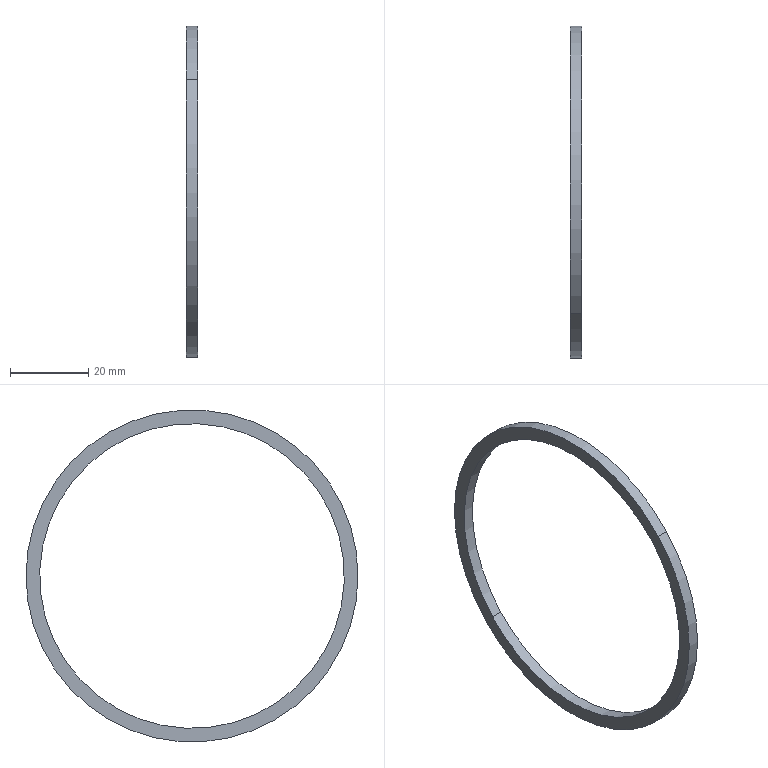Component | SolidWorks | 10BearingLockPlate-1 | 1 solid | 6 faces | box 3 x 85 x 85 mm | volume 2688 mm3 | cylinder 4 | plane 2 | commonest cylinder face diameters 78 x2 85 x2
build123d program:
from build123d import *

# Parameters (mm, degrees)
SKETCH26_R          = 42.5
SKETCH26_R_2        = 39
BOSS_EXTRUDE1_DEPTH = 3


with BuildPart() as part:
    # Sketch26 → Boss-Extrude1 (new body)
    with BuildSketch(Plane.XY):
        Circle(SKETCH26_R)
        Circle(SKETCH26_R_2, mode=Mode.SUBTRACT)
    extrude(amount=BOSS_EXTRUDE1_DEPTH)


solid = part.part

# Placed as in the assembly
solid = solid.moved(Location((210.085, -90.191, 512), (0, 90, 0)))
STEP:
#1=COLOUR_RGB('',0.7922,0.8196,0.9333);
#2=FILL_AREA_STYLE_COLOUR('',#1);
#3=FILL_AREA_STYLE('',(#2));
#4=SURFACE_STYLE_FILL_AREA(#3);
#5=SURFACE_SIDE_STYLE('',(#4));
#6=SURFACE_STYLE_USAGE(.BOTH.,#5);
#7=PRESENTATION_STYLE_ASSIGNMENT((#6));
#8=CARTESIAN_POINT('',(8.271,-2.422,19.117));
#9=VERTEX_POINT('',#8);
#10=CARTESIAN_POINT('',(8.271,-4.68,21.198));
#11=VERTEX_POINT('',#10);
#12=CARTESIAN_POINT('',(8.271,-3.551,20.157));
#13=DIRECTION('',(-1.,0.,0.));
#14=DIRECTION('',(0.,-0.7354,0.6777));
#15=AXIS2_PLACEMENT_3D('',#12,#13,#14);
#16=CIRCLE('',#15,1.535);
#17=EDGE_CURVE('',#9,#11,#16,.T.);
#18=ORIENTED_EDGE('',*,*,#17,.T.);
#19=CARTESIAN_POINT('',(8.389,-4.68,21.198));
#20=VERTEX_POINT('',#19);
#21=CARTESIAN_POINT('',(8.271,-4.68,21.198));
#22=DIRECTION('',(1.,0.,0.));
#23=VECTOR('',#22,39.37);
#24=LINE('',#21,#23);
#25=EDGE_CURVE('',#11,#20,#24,.T.);
#26=ORIENTED_EDGE('',*,*,#25,.T.);
#27=CARTESIAN_POINT('',(8.389,-2.422,19.117));
#28=VERTEX_POINT('',#27);
#29=CARTESIAN_POINT('',(8.389,-3.551,20.157));
#30=DIRECTION('',(-1.,0.,0.));
#31=DIRECTION('',(0.,-0.7354,0.6777));
#32=AXIS2_PLACEMENT_3D('',#29,#30,#31);
#33=CIRCLE('',#32,1.535);
#34=EDGE_CURVE('',#28,#20,#33,.T.);
#35=ORIENTED_EDGE('',*,*,#34,.F.);
#36=CARTESIAN_POINT('',(8.271,-2.422,19.117));
#37=DIRECTION('',(1.,0.,0.));
#38=VECTOR('',#37,39.37);
#39=LINE('',#36,#38);
#40=EDGE_CURVE('',#9,#28,#39,.T.);
#41=ORIENTED_EDGE('',*,*,#40,.F.);
#42=EDGE_LOOP('',(#18,#26,#35,#41));
#43=FACE_OUTER_BOUND('',#42,.T.);
#44=CARTESIAN_POINT('',(8.271,-3.551,20.157));
#45=DIRECTION('',(1.,0.,0.));
#46=DIRECTION('',(0.,0.7354,-0.6777));
#47=AXIS2_PLACEMENT_3D('',#44,#45,#46);
#48=CYLINDRICAL_SURFACE('',#47,1.535);
#49=ADVANCED_FACE('',(#43),#48,.F.);
#50=CARTESIAN_POINT('',(8.271,-4.781,21.291));
#51=VERTEX_POINT('',#50);
#52=CARTESIAN_POINT('',(8.271,-2.32,19.024));
#53=VERTEX_POINT('',#52);
#54=CARTESIAN_POINT('',(8.271,-3.551,20.157));
#55=DIRECTION('',(-1.,0.,0.));
#56=DIRECTION('',(0.,-0.7354,0.6777));
#57=AXIS2_PLACEMENT_3D('',#54,#55,#56);
#58=CIRCLE('',#57,1.673);
#59=EDGE_CURVE('',#51,#53,#58,.T.);
#60=ORIENTED_EDGE('',*,*,#59,.F.);
#61=CARTESIAN_POINT('',(8.389,-4.781,21.291));
#62=VERTEX_POINT('',#61);
#63=CARTESIAN_POINT('',(8.271,-4.781,21.291));
#64=DIRECTION('',(1.,0.,0.));
#65=VECTOR('',#64,39.37);
#66=LINE('',#63,#65);
#67=EDGE_CURVE('',#51,#62,#66,.T.);
#68=ORIENTED_EDGE('',*,*,#67,.T.);
#69=CARTESIAN_POINT('',(8.389,-2.32,19.024));
#70=VERTEX_POINT('',#69);
#71=CARTESIAN_POINT('',(8.389,-3.551,20.157));
#72=DIRECTION('',(-1.,0.,0.));
#73=DIRECTION('',(0.,-0.7354,0.6777));
#74=AXIS2_PLACEMENT_3D('',#71,#72,#73);
#75=CIRCLE('',#74,1.673);
#76=EDGE_CURVE('',#62,#70,#75,.T.);
#77=ORIENTED_EDGE('',*,*,#76,.T.);
#78=CARTESIAN_POINT('',(8.271,-2.32,19.024));
#79=DIRECTION('',(1.,0.,0.));
#80=VECTOR('',#79,39.37);
#81=LINE('',#78,#80);
#82=EDGE_CURVE('',#53,#70,#81,.T.);
#83=ORIENTED_EDGE('',*,*,#82,.F.);
#84=EDGE_LOOP('',(#60,#68,#77,#83));
#85=FACE_OUTER_BOUND('',#84,.T.);
#86=CARTESIAN_POINT('',(8.271,-3.551,20.157));
#87=DIRECTION('',(1.,0.,0.));
#88=DIRECTION('',(0.,0.7354,-0.6777));
#89=AXIS2_PLACEMENT_3D('',#86,#87,#88);
#90=CYLINDRICAL_SURFACE('',#89,1.673);
#91=ADVANCED_FACE('',(#85),#90,.T.);
#92=CARTESIAN_POINT('',(8.271,-3.551,20.157));
#93=DIRECTION('',(-1.,0.,0.));
#94=DIRECTION('',(0.,-0.7354,0.6777));
#95=AXIS2_PLACEMENT_3D('',#92,#93,#94);
#96=CIRCLE('',#95,1.673);
#97=EDGE_CURVE('',#53,#51,#96,.T.);
#98=ORIENTED_EDGE('',*,*,#97,.T.);
#99=ORIENTED_EDGE('',*,*,#59,.T.);
#100=EDGE_LOOP('',(#98,#99));
#101=FACE_OUTER_BOUND('',#100,.T.);
#102=ORIENTED_EDGE('',*,*,#17,.F.);
#103=CARTESIAN_POINT('',(8.271,-3.551,20.157));
#104=DIRECTION('',(-1.,0.,0.));
#105=DIRECTION('',(0.,-0.7354,0.6777));
#106=AXIS2_PLACEMENT_3D('',#103,#104,#105);
#107=CIRCLE('',#106,1.535);
#108=EDGE_CURVE('',#11,#9,#107,.T.);
#109=ORIENTED_EDGE('',*,*,#108,.F.);
#110=EDGE_LOOP('',(#102,#109));
#111=FACE_BOUND('',#110,.T.);
#112=CARTESIAN_POINT('',(8.271,-3.551,20.157));
#113=DIRECTION('',(-1.,0.,0.));
#114=DIRECTION('',(0.,-0.7354,0.6777));
#115=AXIS2_PLACEMENT_3D('',#112,#113,#114);
#116=PLANE('',#115);
#117=ADVANCED_FACE('',(#101,#111),#116,.T.);
#118=CARTESIAN_POINT('',(8.389,-3.551,20.157));
#119=DIRECTION('',(-1.,0.,0.));
#120=DIRECTION('',(0.,-0.7354,0.6777));
#121=AXIS2_PLACEMENT_3D('',#118,#119,#120);
#122=CIRCLE('',#121,1.673);
#123=EDGE_CURVE('',#70,#62,#122,.T.);
#124=ORIENTED_EDGE('',*,*,#123,.F.);
#125=ORIENTED_EDGE('',*,*,#76,.F.);
#126=EDGE_LOOP('',(#124,#125));
#127=FACE_OUTER_BOUND('',#126,.T.);
#128=ORIENTED_EDGE('',*,*,#34,.T.);
#129=CARTESIAN_POINT('',(8.389,-3.551,20.157));
#130=DIRECTION('',(-1.,0.,0.));
#131=DIRECTION('',(0.,-0.7354,0.6777));
#132=AXIS2_PLACEMENT_3D('',#129,#130,#131);
#133=CIRCLE('',#132,1.535);
#134=EDGE_CURVE('',#20,#28,#133,.T.);
#135=ORIENTED_EDGE('',*,*,#134,.T.);
#136=EDGE_LOOP('',(#128,#135));
#137=FACE_BOUND('',#136,.T.);
#138=CARTESIAN_POINT('',(8.389,-3.551,20.157));
#139=DIRECTION('',(-1.,0.,0.));
#140=DIRECTION('',(0.,-0.7354,0.6777));
#141=AXIS2_PLACEMENT_3D('',#138,#139,#140);
#142=PLANE('',#141);
#143=ADVANCED_FACE('',(#127,#137),#142,.F.);
#144=ORIENTED_EDGE('',*,*,#67,.F.);
#145=ORIENTED_EDGE('',*,*,#97,.F.);
#146=ORIENTED_EDGE('',*,*,#82,.T.);
#147=ORIENTED_EDGE('',*,*,#123,.T.);
#148=EDGE_LOOP('',(#144,#145,#146,#147));
#149=FACE_OUTER_BOUND('',#148,.T.);
#150=CARTESIAN_POINT('',(8.271,-3.551,20.157));
#151=DIRECTION('',(1.,0.,0.));
#152=DIRECTION('',(0.,0.7354,-0.6777));
#153=AXIS2_PLACEMENT_3D('',#150,#151,#152);
#154=CYLINDRICAL_SURFACE('',#153,1.673);
#155=ADVANCED_FACE('',(#149),#154,.T.);
#156=ORIENTED_EDGE('',*,*,#25,.F.);
#157=ORIENTED_EDGE('',*,*,#108,.T.);
#158=ORIENTED_EDGE('',*,*,#40,.T.);
#159=ORIENTED_EDGE('',*,*,#134,.F.);
#160=EDGE_LOOP('',(#156,#157,#158,#159));
#161=FACE_OUTER_BOUND('',#160,.T.);
#162=CARTESIAN_POINT('',(8.271,-3.551,20.157));
#163=DIRECTION('',(1.,0.,0.));
#164=DIRECTION('',(0.,0.7354,-0.6777));
#165=AXIS2_PLACEMENT_3D('',#162,#163,#164);
#166=CYLINDRICAL_SURFACE('',#165,1.535);
#167=ADVANCED_FACE('',(#161),#166,.F.);
#168=CLOSED_SHELL('',(#49,#91,#117,#143,#155,#167));
#169=MANIFOLD_SOLID_BREP('',#168);
#170=STYLED_ITEM('',(#7),#169);
#171=(LENGTH_UNIT()NAMED_UNIT(*)SI_UNIT($,.METRE.));
#172=LENGTH_MEASURE_WITH_UNIT(LENGTH_MEASURE(0.0254),#171);
#173=DIMENSIONAL_EXPONENTS(1.,0.,0.,0.,0.,0.,0.);
#174=(CONVERSION_BASED_UNIT('',#172)LENGTH_UNIT()NAMED_UNIT(#173));
#175=UNCERTAINTY_MEASURE_WITH_UNIT(LENGTH_MEASURE(0.00001),#174,'','');
#176=(NAMED_UNIT(*)PLANE_ANGLE_UNIT()SI_UNIT($,.RADIAN.));
#177=(NAMED_UNIT(*)SI_UNIT($,.STERADIAN.)SOLID_ANGLE_UNIT());
#178=(GEOMETRIC_REPRESENTATION_CONTEXT(3)GLOBAL_UNCERTAINTY_ASSIGNED_CONTEXT((#175))GLOBAL_UNIT_ASSIGNED_CONTEXT((#174,#176,#177))REPRESENTATION_CONTEXT('',''));
#179=MECHANICAL_DESIGN_GEOMETRIC_PRESENTATION_REPRESENTATION('',(#170),#178);
#180=CARTESIAN_POINT('',(0.,0.,0.));
#181=DIRECTION('',(0.,0.,1.));
#182=DIRECTION('',(1.,0.,0.));
#183=AXIS2_PLACEMENT_3D('',#180,#181,#182);
#184=(LENGTH_UNIT()NAMED_UNIT(*)SI_UNIT($,.METRE.));
#185=LENGTH_MEASURE_WITH_UNIT(LENGTH_MEASURE(0.0254),#184);
#186=DIMENSIONAL_EXPONENTS(1.,0.,0.,0.,0.,0.,0.);
#187=(CONVERSION_BASED_UNIT('',#185)LENGTH_UNIT()NAMED_UNIT(#186));
#188=UNCERTAINTY_MEASURE_WITH_UNIT(LENGTH_MEASURE(0.00001),#187,'','');
#189=(NAMED_UNIT(*)PLANE_ANGLE_UNIT()SI_UNIT($,.RADIAN.));
#190=(NAMED_UNIT(*)SI_UNIT($,.STERADIAN.)SOLID_ANGLE_UNIT());
#191=(GEOMETRIC_REPRESENTATION_CONTEXT(3)GLOBAL_UNCERTAINTY_ASSIGNED_CONTEXT((#188))GLOBAL_UNIT_ASSIGNED_CONTEXT((#187,#189,#190))REPRESENTATION_CONTEXT('',''));
#192=ADVANCED_BREP_SHAPE_REPRESENTATION('',(#169,#183),#191);
#193=PRESENTATION_LAYER_ASSIGNMENT('','',(#170));